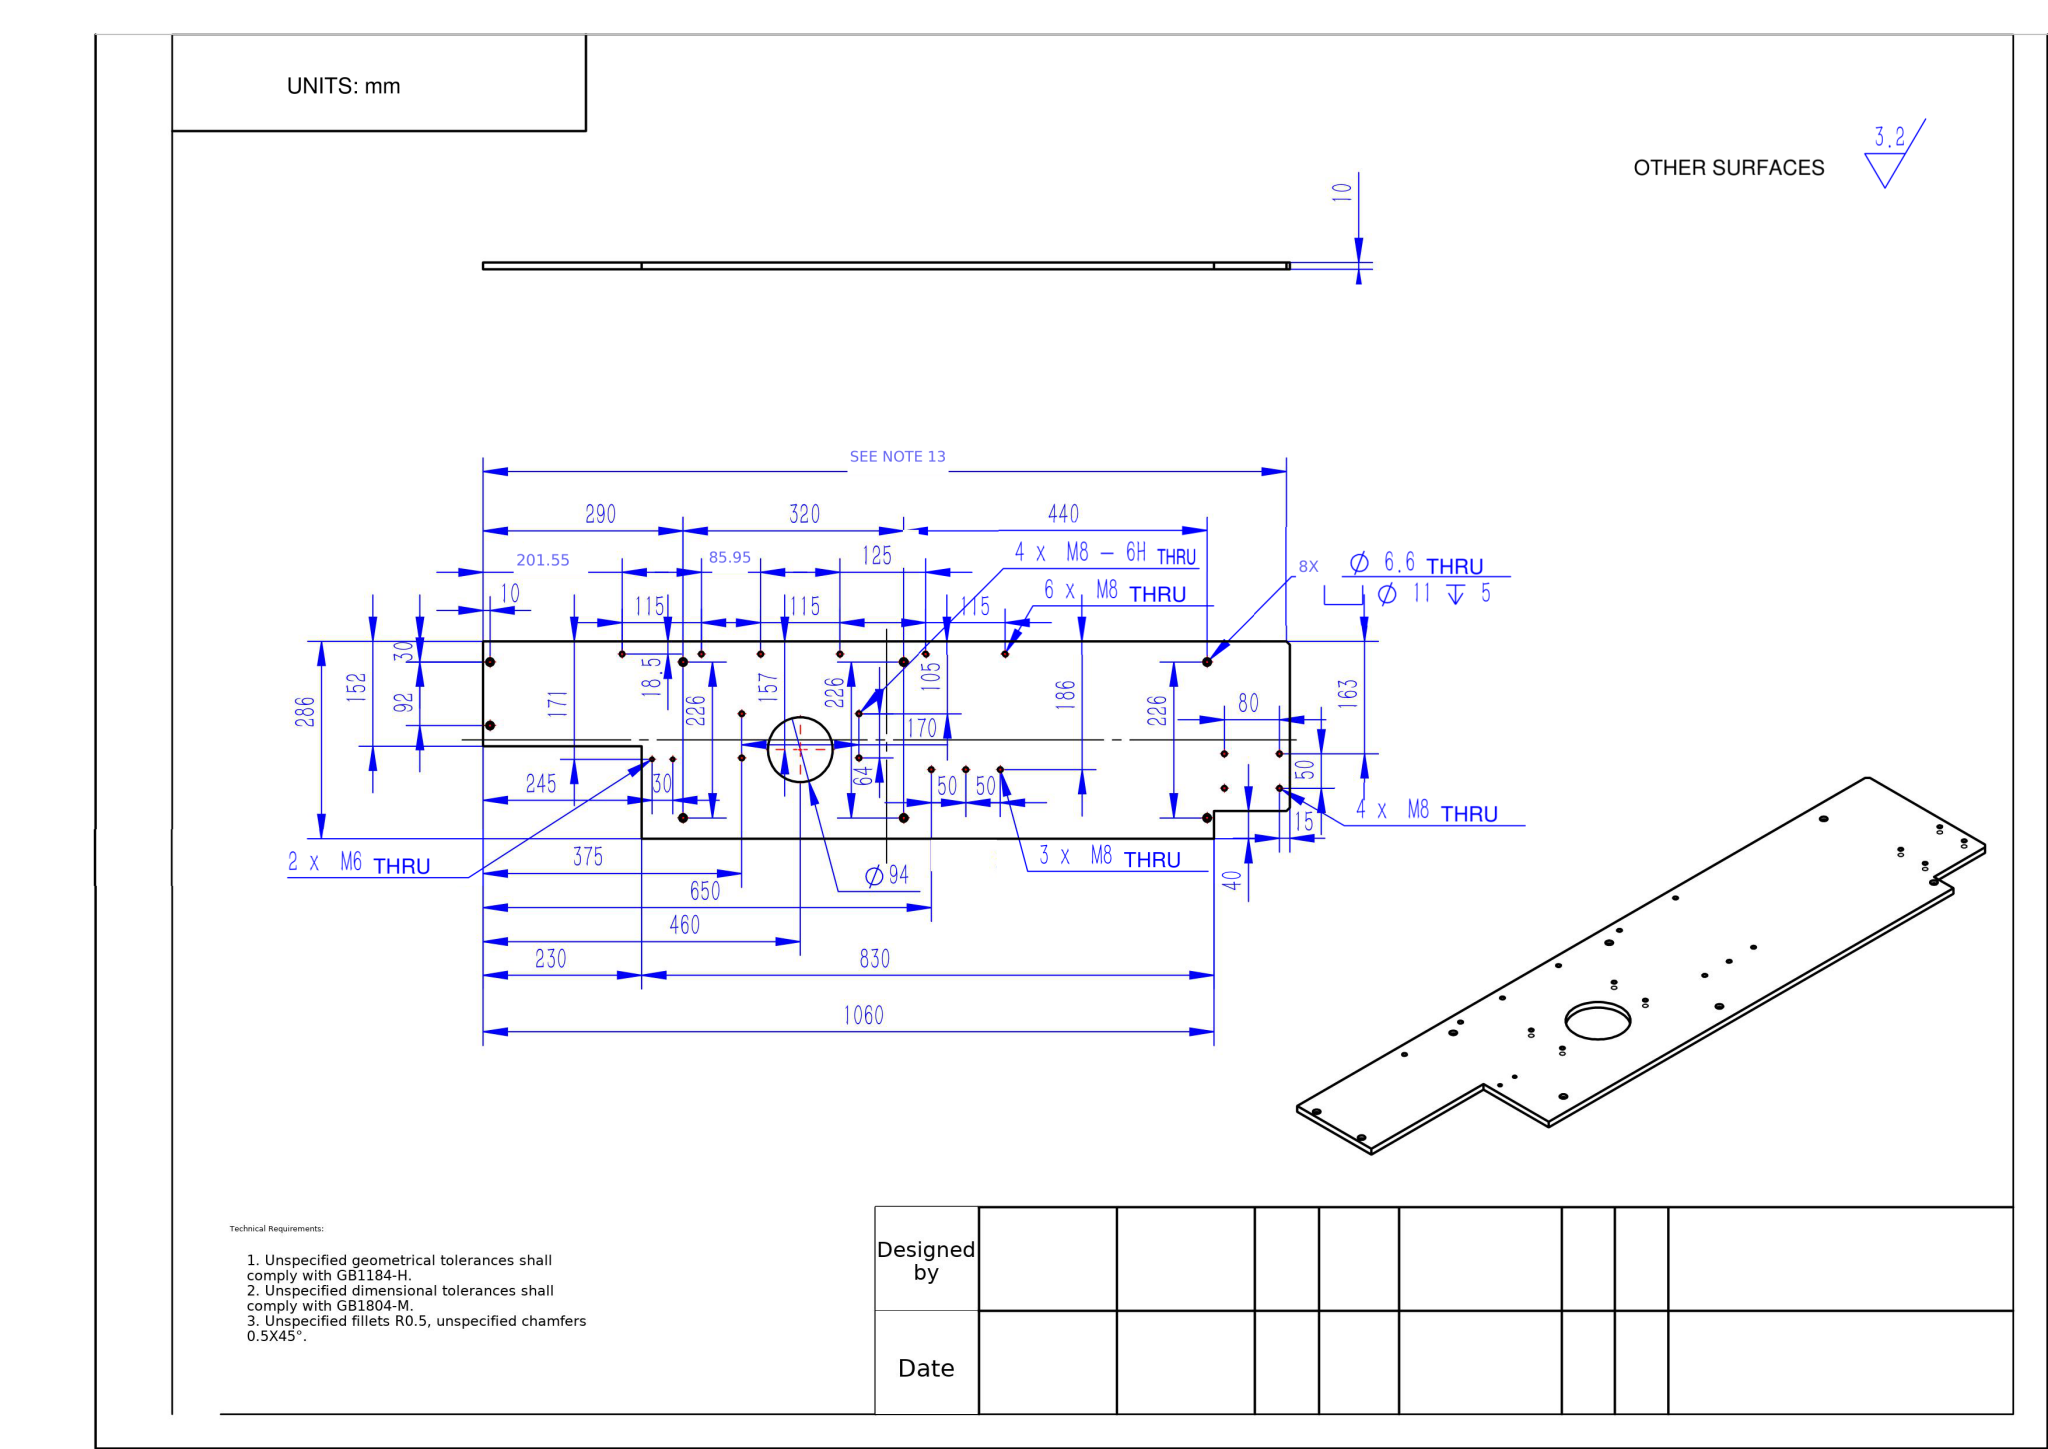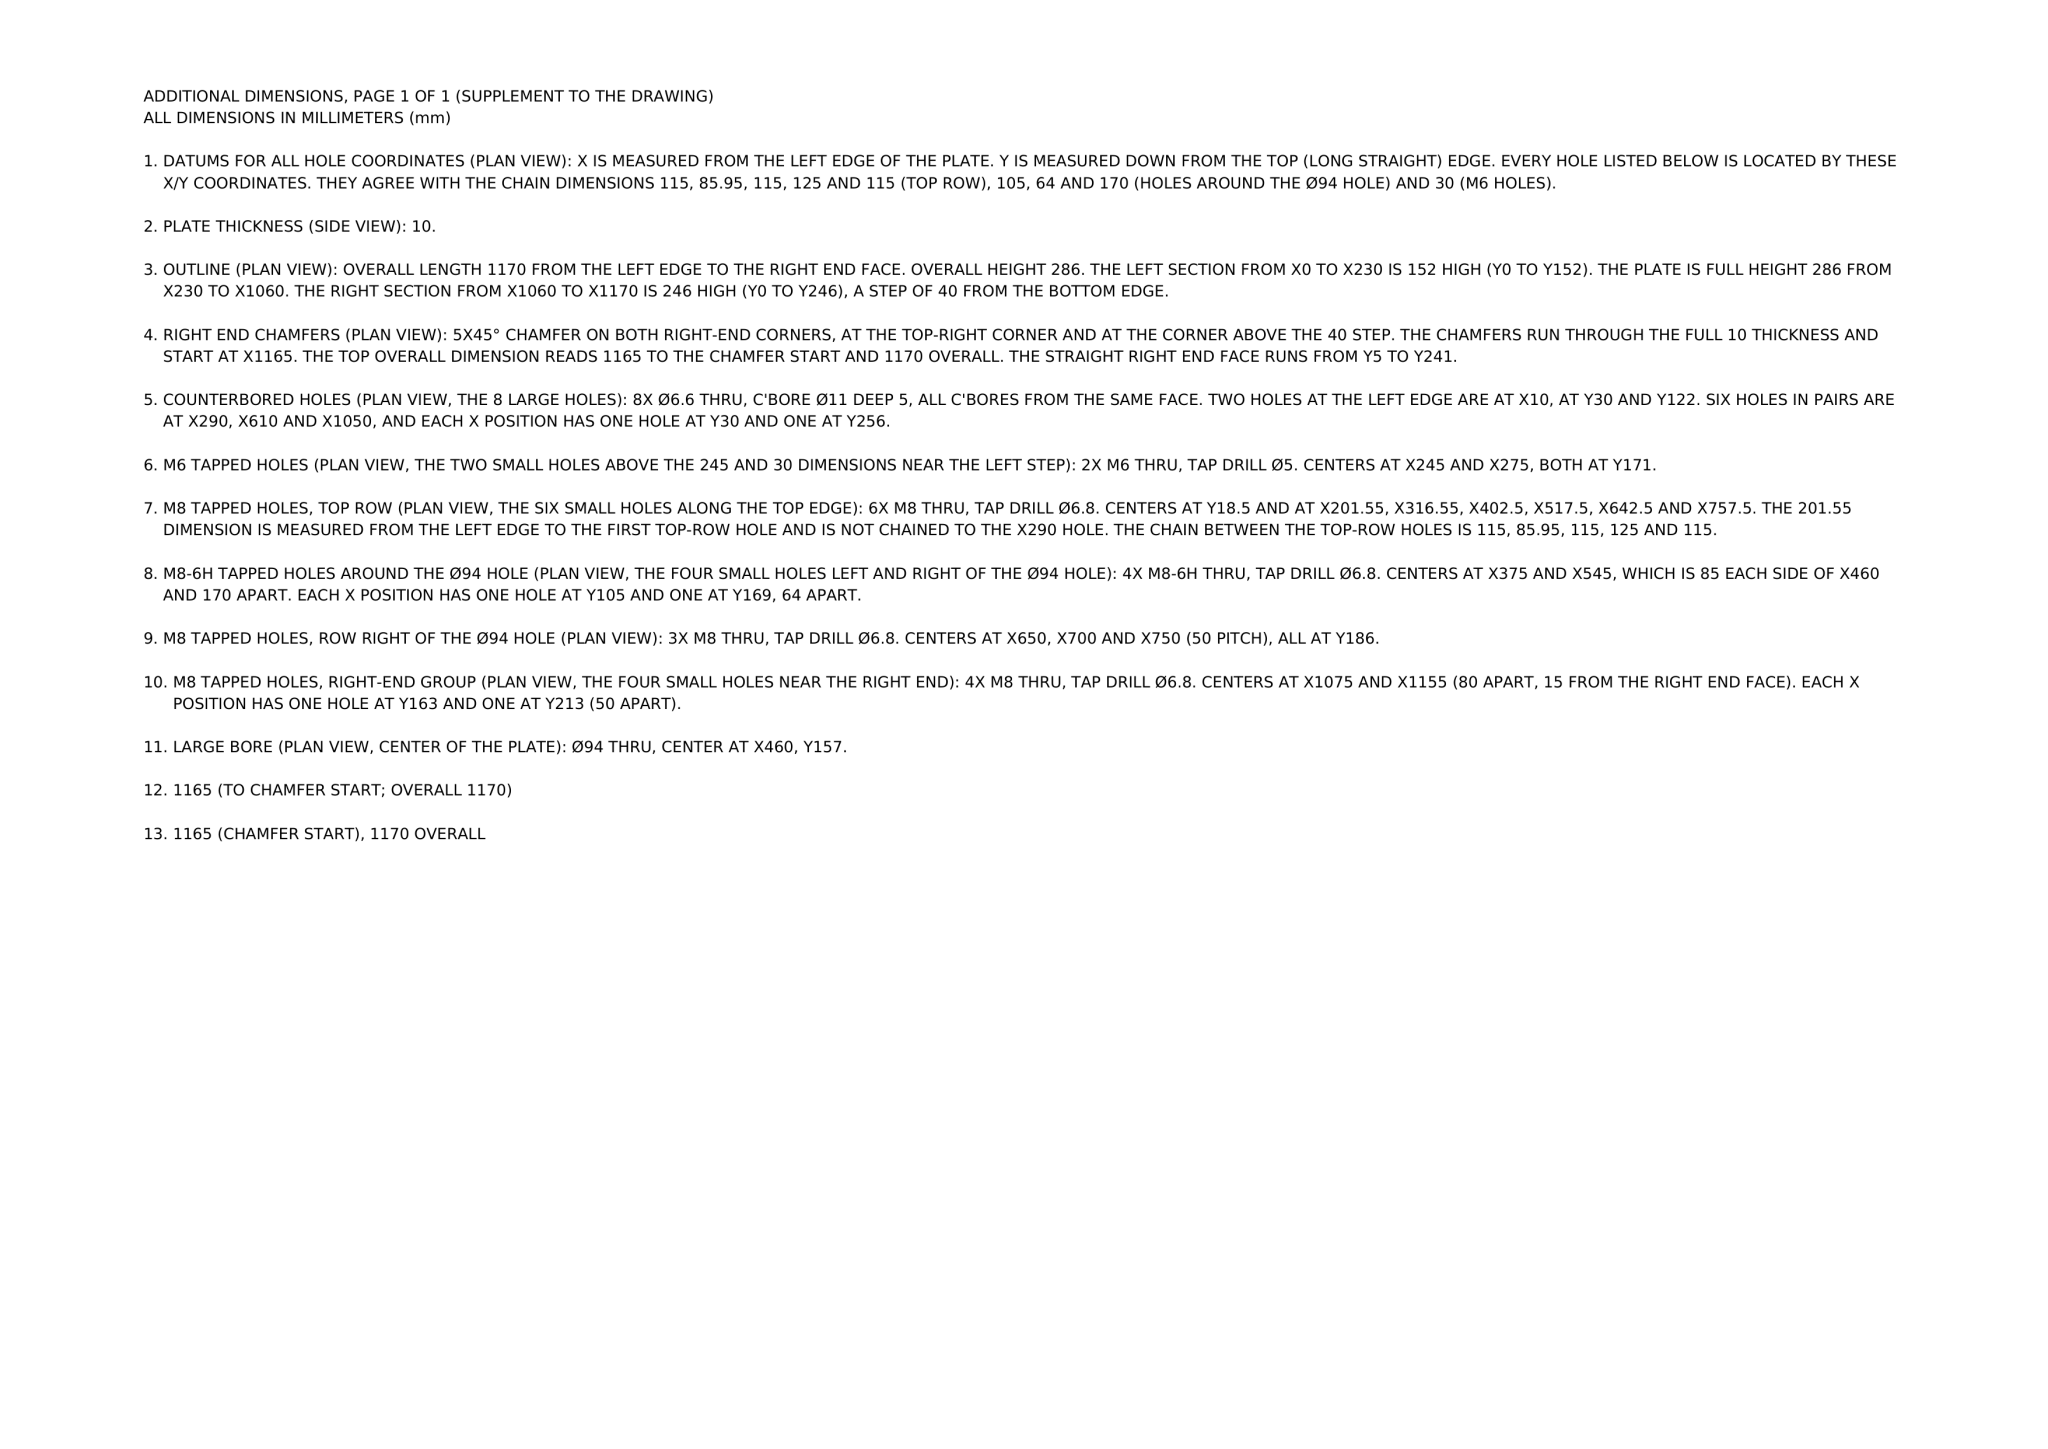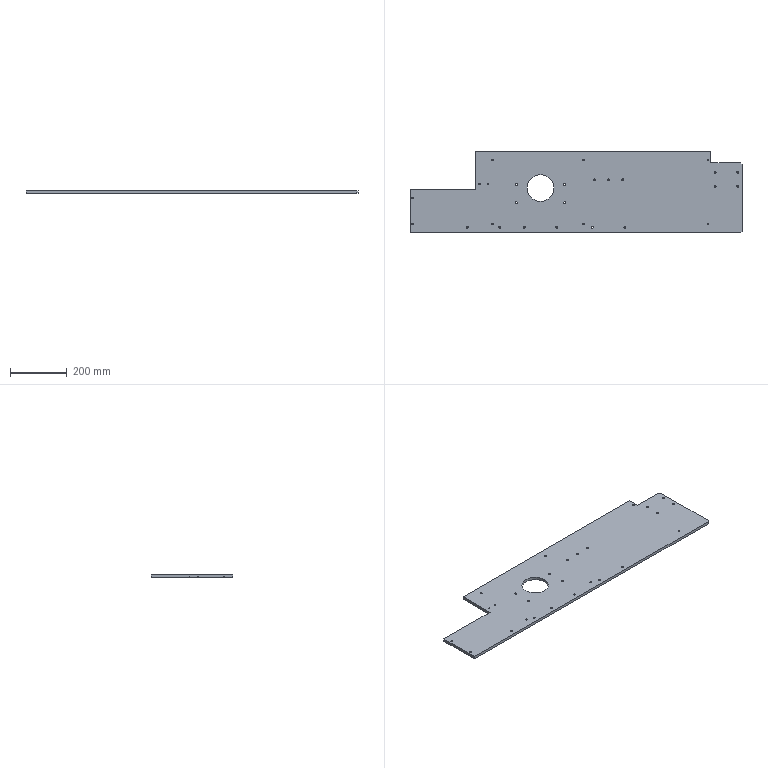Part | NX | mm | 1 solid | 92 faces | box 1170 x 286 x 10 mm | volume 2912616 mm3 | cylinder 72 | plane 20 | commonest cylinder face diameters 6.8 x34 11 x16 6.6 x16 5 x4 94 x2